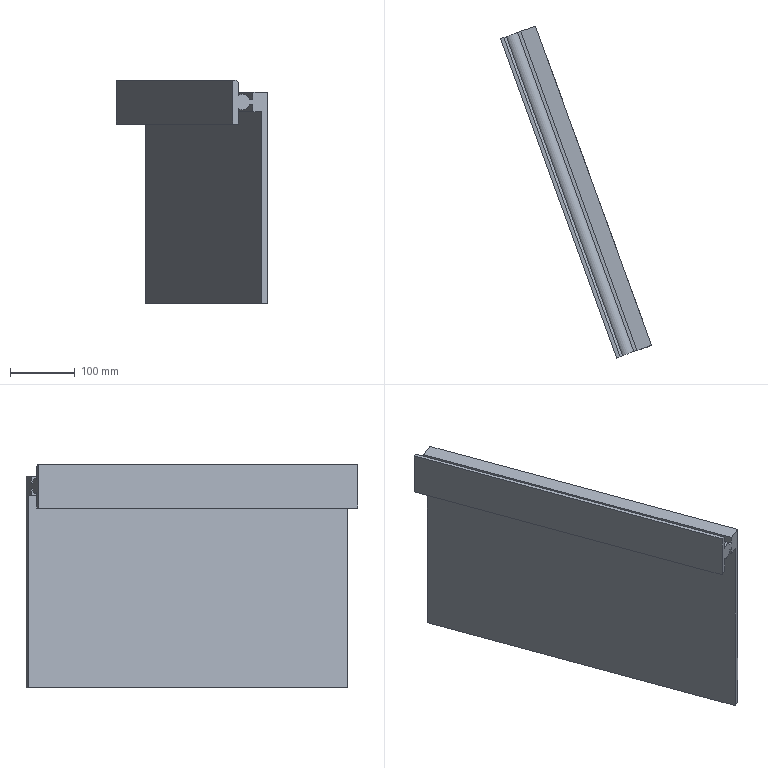Component | NX | PART_2 | 1 solid | 79 faces | volume 2403630 mm3 | plane 77 | cylinder 2 | commonest cylinder face diameters 24 x2